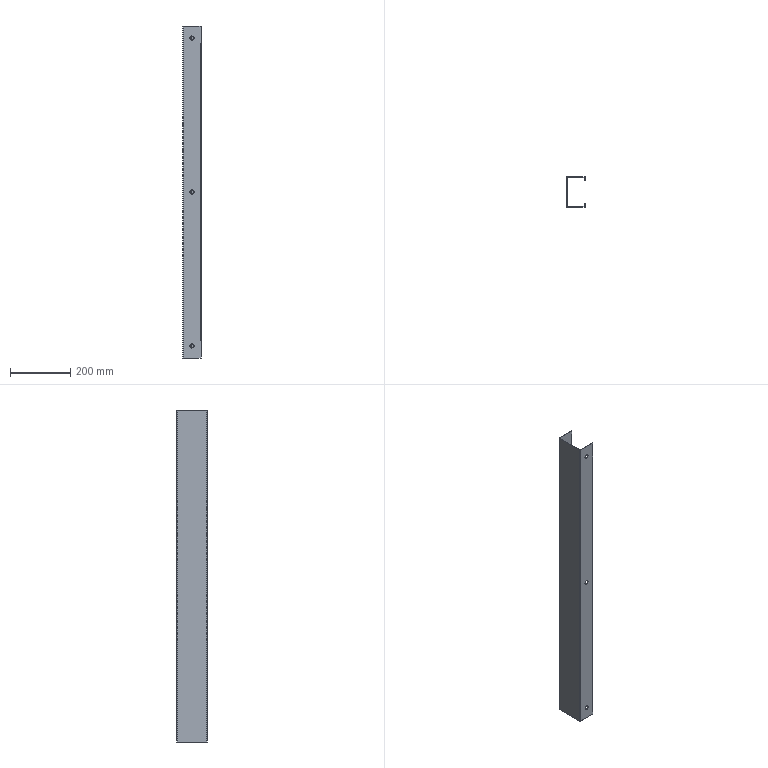Component | SolidWorks | BaseWeldment-1_BottomFrameFront-1 | 1 solid | 64 faces | volume 385728 mm3 | cylinder 30 | plane 30 | spline 4 | commonest cylinder face diameters 4 x10 14 x6 8.5 x6 0.2 x4 3.2 x4